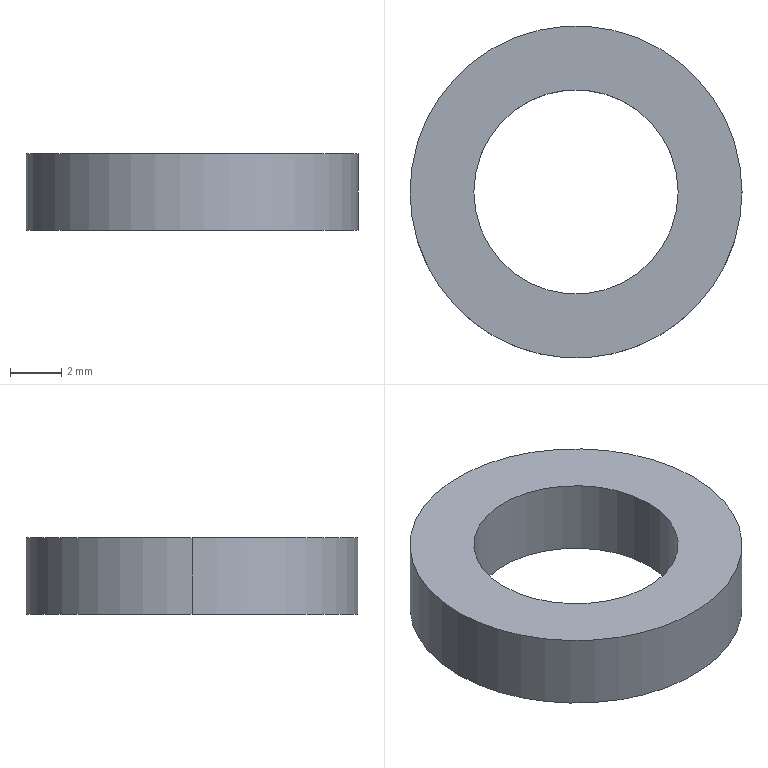Component | SolidWorks | 75-02-27ConnectingRodSpacer-1 | 1 solid | 6 faces | box 13 x 13 x 3 mm | volume 247 mm3 | cylinder 4 | plane 2 | commonest cylinder face diameters 8 x2 13 x2 | material A3 Steel
build123d program:
from build123d import *

# Parameters (mm, degrees)
SKETCH1_R           = 6.5
SKETCH1_R_2         = 4
BOSS_EXTRUDE1_DEPTH = 3


with BuildPart() as part:
    # Sketch1 → Boss-Extrude1 (new body)
    with BuildSketch(Plane.XY):
        Circle(SKETCH1_R)
        Circle(SKETCH1_R_2, mode=Mode.SUBTRACT)
    extrude(amount=BOSS_EXTRUDE1_DEPTH)


solid = part.part

# Placed as in the assembly
solid = solid.moved(Location((-16.556, 86.857, 63.25), (0, 0, 0)))
STEP:
#1=COLOUR_RGB('',0.7922,0.8196,0.9333);
#2=FILL_AREA_STYLE_COLOUR('',#1);
#3=FILL_AREA_STYLE('',(#2));
#4=SURFACE_STYLE_FILL_AREA(#3);
#5=SURFACE_SIDE_STYLE('',(#4));
#6=SURFACE_STYLE_USAGE(.BOTH.,#5);
#7=PRESENTATION_STYLE_ASSIGNMENT((#6));
#8=CARTESIAN_POINT('',(-0.8093,3.42,2.608));
#9=VERTEX_POINT('',#8);
#10=CARTESIAN_POINT('',(-0.4943,3.42,2.608));
#11=VERTEX_POINT('',#10);
#12=CARTESIAN_POINT('',(-0.6518,3.42,2.608));
#13=DIRECTION('',(0.,0.,1.));
#14=DIRECTION('',(1.,0.,0.));
#15=AXIS2_PLACEMENT_3D('',#12,#13,#14);
#16=CIRCLE('',#15,0.1575);
#17=EDGE_CURVE('',#9,#11,#16,.T.);
#18=ORIENTED_EDGE('',*,*,#17,.T.);
#19=CARTESIAN_POINT('',(-0.4943,3.42,2.49));
#20=VERTEX_POINT('',#19);
#21=CARTESIAN_POINT('',(-0.4943,3.42,2.608));
#22=DIRECTION('',(0.,0.,-1.));
#23=VECTOR('',#22,39.37);
#24=LINE('',#21,#23);
#25=EDGE_CURVE('',#11,#20,#24,.T.);
#26=ORIENTED_EDGE('',*,*,#25,.T.);
#27=CARTESIAN_POINT('',(-0.8093,3.42,2.49));
#28=VERTEX_POINT('',#27);
#29=CARTESIAN_POINT('',(-0.6518,3.42,2.49));
#30=DIRECTION('',(0.,0.,1.));
#31=DIRECTION('',(1.,0.,0.));
#32=AXIS2_PLACEMENT_3D('',#29,#30,#31);
#33=CIRCLE('',#32,0.1575);
#34=EDGE_CURVE('',#28,#20,#33,.T.);
#35=ORIENTED_EDGE('',*,*,#34,.F.);
#36=CARTESIAN_POINT('',(-0.8093,3.42,2.608));
#37=DIRECTION('',(0.,0.,-1.));
#38=VECTOR('',#37,39.37);
#39=LINE('',#36,#38);
#40=EDGE_CURVE('',#9,#28,#39,.T.);
#41=ORIENTED_EDGE('',*,*,#40,.F.);
#42=EDGE_LOOP('',(#18,#26,#35,#41));
#43=FACE_OUTER_BOUND('',#42,.T.);
#44=CARTESIAN_POINT('',(-0.6518,3.42,2.608));
#45=DIRECTION('',(0.,0.,-1.));
#46=DIRECTION('',(-1.,0.,0.));
#47=AXIS2_PLACEMENT_3D('',#44,#45,#46);
#48=CYLINDRICAL_SURFACE('',#47,0.1575);
#49=ADVANCED_FACE('',(#43),#48,.F.);
#50=CARTESIAN_POINT('',(-0.3959,3.42,2.608));
#51=VERTEX_POINT('',#50);
#52=CARTESIAN_POINT('',(-0.9077,3.42,2.608));
#53=VERTEX_POINT('',#52);
#54=CARTESIAN_POINT('',(-0.6518,3.42,2.608));
#55=DIRECTION('',(0.,0.,1.));
#56=DIRECTION('',(1.,0.,0.));
#57=AXIS2_PLACEMENT_3D('',#54,#55,#56);
#58=CIRCLE('',#57,0.2559);
#59=EDGE_CURVE('',#51,#53,#58,.T.);
#60=ORIENTED_EDGE('',*,*,#59,.F.);
#61=CARTESIAN_POINT('',(-0.3959,3.42,2.49));
#62=VERTEX_POINT('',#61);
#63=CARTESIAN_POINT('',(-0.3959,3.42,2.608));
#64=DIRECTION('',(0.,0.,-1.));
#65=VECTOR('',#64,39.37);
#66=LINE('',#63,#65);
#67=EDGE_CURVE('',#51,#62,#66,.T.);
#68=ORIENTED_EDGE('',*,*,#67,.T.);
#69=CARTESIAN_POINT('',(-0.9077,3.42,2.49));
#70=VERTEX_POINT('',#69);
#71=CARTESIAN_POINT('',(-0.6518,3.42,2.49));
#72=DIRECTION('',(0.,0.,1.));
#73=DIRECTION('',(1.,0.,0.));
#74=AXIS2_PLACEMENT_3D('',#71,#72,#73);
#75=CIRCLE('',#74,0.2559);
#76=EDGE_CURVE('',#62,#70,#75,.T.);
#77=ORIENTED_EDGE('',*,*,#76,.T.);
#78=CARTESIAN_POINT('',(-0.9077,3.42,2.608));
#79=DIRECTION('',(0.,0.,-1.));
#80=VECTOR('',#79,39.37);
#81=LINE('',#78,#80);
#82=EDGE_CURVE('',#53,#70,#81,.T.);
#83=ORIENTED_EDGE('',*,*,#82,.F.);
#84=EDGE_LOOP('',(#60,#68,#77,#83));
#85=FACE_OUTER_BOUND('',#84,.T.);
#86=CARTESIAN_POINT('',(-0.6518,3.42,2.608));
#87=DIRECTION('',(0.,0.,-1.));
#88=DIRECTION('',(-1.,0.,0.));
#89=AXIS2_PLACEMENT_3D('',#86,#87,#88);
#90=CYLINDRICAL_SURFACE('',#89,0.2559);
#91=ADVANCED_FACE('',(#85),#90,.T.);
#92=CARTESIAN_POINT('',(-0.6518,3.42,2.608));
#93=DIRECTION('',(0.,0.,1.));
#94=DIRECTION('',(1.,0.,0.));
#95=AXIS2_PLACEMENT_3D('',#92,#93,#94);
#96=CIRCLE('',#95,0.2559);
#97=EDGE_CURVE('',#53,#51,#96,.T.);
#98=ORIENTED_EDGE('',*,*,#97,.T.);
#99=ORIENTED_EDGE('',*,*,#59,.T.);
#100=EDGE_LOOP('',(#98,#99));
#101=FACE_OUTER_BOUND('',#100,.T.);
#102=ORIENTED_EDGE('',*,*,#17,.F.);
#103=CARTESIAN_POINT('',(-0.6518,3.42,2.608));
#104=DIRECTION('',(0.,0.,1.));
#105=DIRECTION('',(1.,0.,0.));
#106=AXIS2_PLACEMENT_3D('',#103,#104,#105);
#107=CIRCLE('',#106,0.1575);
#108=EDGE_CURVE('',#11,#9,#107,.T.);
#109=ORIENTED_EDGE('',*,*,#108,.F.);
#110=EDGE_LOOP('',(#102,#109));
#111=FACE_BOUND('',#110,.T.);
#112=CARTESIAN_POINT('',(-0.6518,3.42,2.608));
#113=DIRECTION('',(0.,0.,1.));
#114=DIRECTION('',(1.,0.,0.));
#115=AXIS2_PLACEMENT_3D('',#112,#113,#114);
#116=PLANE('',#115);
#117=ADVANCED_FACE('',(#101,#111),#116,.T.);
#118=CARTESIAN_POINT('',(-0.6518,3.42,2.49));
#119=DIRECTION('',(0.,0.,1.));
#120=DIRECTION('',(1.,0.,0.));
#121=AXIS2_PLACEMENT_3D('',#118,#119,#120);
#122=CIRCLE('',#121,0.2559);
#123=EDGE_CURVE('',#70,#62,#122,.T.);
#124=ORIENTED_EDGE('',*,*,#123,.F.);
#125=ORIENTED_EDGE('',*,*,#76,.F.);
#126=EDGE_LOOP('',(#124,#125));
#127=FACE_OUTER_BOUND('',#126,.T.);
#128=ORIENTED_EDGE('',*,*,#34,.T.);
#129=CARTESIAN_POINT('',(-0.6518,3.42,2.49));
#130=DIRECTION('',(0.,0.,1.));
#131=DIRECTION('',(1.,0.,0.));
#132=AXIS2_PLACEMENT_3D('',#129,#130,#131);
#133=CIRCLE('',#132,0.1575);
#134=EDGE_CURVE('',#20,#28,#133,.T.);
#135=ORIENTED_EDGE('',*,*,#134,.T.);
#136=EDGE_LOOP('',(#128,#135));
#137=FACE_BOUND('',#136,.T.);
#138=CARTESIAN_POINT('',(-0.6518,3.42,2.49));
#139=DIRECTION('',(0.,0.,1.));
#140=DIRECTION('',(1.,0.,0.));
#141=AXIS2_PLACEMENT_3D('',#138,#139,#140);
#142=PLANE('',#141);
#143=ADVANCED_FACE('',(#127,#137),#142,.F.);
#144=ORIENTED_EDGE('',*,*,#67,.F.);
#145=ORIENTED_EDGE('',*,*,#97,.F.);
#146=ORIENTED_EDGE('',*,*,#82,.T.);
#147=ORIENTED_EDGE('',*,*,#123,.T.);
#148=EDGE_LOOP('',(#144,#145,#146,#147));
#149=FACE_OUTER_BOUND('',#148,.T.);
#150=CARTESIAN_POINT('',(-0.6518,3.42,2.608));
#151=DIRECTION('',(0.,0.,-1.));
#152=DIRECTION('',(-1.,0.,0.));
#153=AXIS2_PLACEMENT_3D('',#150,#151,#152);
#154=CYLINDRICAL_SURFACE('',#153,0.2559);
#155=ADVANCED_FACE('',(#149),#154,.T.);
#156=ORIENTED_EDGE('',*,*,#25,.F.);
#157=ORIENTED_EDGE('',*,*,#108,.T.);
#158=ORIENTED_EDGE('',*,*,#40,.T.);
#159=ORIENTED_EDGE('',*,*,#134,.F.);
#160=EDGE_LOOP('',(#156,#157,#158,#159));
#161=FACE_OUTER_BOUND('',#160,.T.);
#162=CARTESIAN_POINT('',(-0.6518,3.42,2.608));
#163=DIRECTION('',(0.,0.,-1.));
#164=DIRECTION('',(-1.,0.,0.));
#165=AXIS2_PLACEMENT_3D('',#162,#163,#164);
#166=CYLINDRICAL_SURFACE('',#165,0.1575);
#167=ADVANCED_FACE('',(#161),#166,.F.);
#168=CLOSED_SHELL('',(#49,#91,#117,#143,#155,#167));
#169=MANIFOLD_SOLID_BREP('',#168);
#170=STYLED_ITEM('',(#7),#169);
#171=PRESENTATION_LAYER_ASSIGNMENT('','',(#170));
#172=(LENGTH_UNIT()NAMED_UNIT(*)SI_UNIT($,.METRE.));
#173=LENGTH_MEASURE_WITH_UNIT(LENGTH_MEASURE(0.0254),#172);
#174=DIMENSIONAL_EXPONENTS(1.,0.,0.,0.,0.,0.,0.);
#175=(CONVERSION_BASED_UNIT('',#173)LENGTH_UNIT()NAMED_UNIT(#174));
#176=UNCERTAINTY_MEASURE_WITH_UNIT(LENGTH_MEASURE(0.00001),#175,'','');
#177=(NAMED_UNIT(*)PLANE_ANGLE_UNIT()SI_UNIT($,.RADIAN.));
#178=(NAMED_UNIT(*)SI_UNIT($,.STERADIAN.)SOLID_ANGLE_UNIT());
#179=(GEOMETRIC_REPRESENTATION_CONTEXT(3)GLOBAL_UNCERTAINTY_ASSIGNED_CONTEXT((#176))GLOBAL_UNIT_ASSIGNED_CONTEXT((#175,#177,#178))REPRESENTATION_CONTEXT('',''));
#180=MECHANICAL_DESIGN_GEOMETRIC_PRESENTATION_REPRESENTATION('',(#170),#179);
#181=CARTESIAN_POINT('',(0.,0.,0.));
#182=DIRECTION('',(0.,0.,1.));
#183=DIRECTION('',(1.,0.,0.));
#184=AXIS2_PLACEMENT_3D('',#181,#182,#183);
#185=(LENGTH_UNIT()NAMED_UNIT(*)SI_UNIT($,.METRE.));
#186=LENGTH_MEASURE_WITH_UNIT(LENGTH_MEASURE(0.0254),#185);
#187=DIMENSIONAL_EXPONENTS(1.,0.,0.,0.,0.,0.,0.);
#188=(CONVERSION_BASED_UNIT('',#186)LENGTH_UNIT()NAMED_UNIT(#187));
#189=UNCERTAINTY_MEASURE_WITH_UNIT(LENGTH_MEASURE(0.00001),#188,'','');
#190=(NAMED_UNIT(*)PLANE_ANGLE_UNIT()SI_UNIT($,.RADIAN.));
#191=(NAMED_UNIT(*)SI_UNIT($,.STERADIAN.)SOLID_ANGLE_UNIT());
#192=(GEOMETRIC_REPRESENTATION_CONTEXT(3)GLOBAL_UNCERTAINTY_ASSIGNED_CONTEXT((#189))GLOBAL_UNIT_ASSIGNED_CONTEXT((#188,#190,#191))REPRESENTATION_CONTEXT('',''));
#193=ADVANCED_BREP_SHAPE_REPRESENTATION('',(#169,#184),#192);